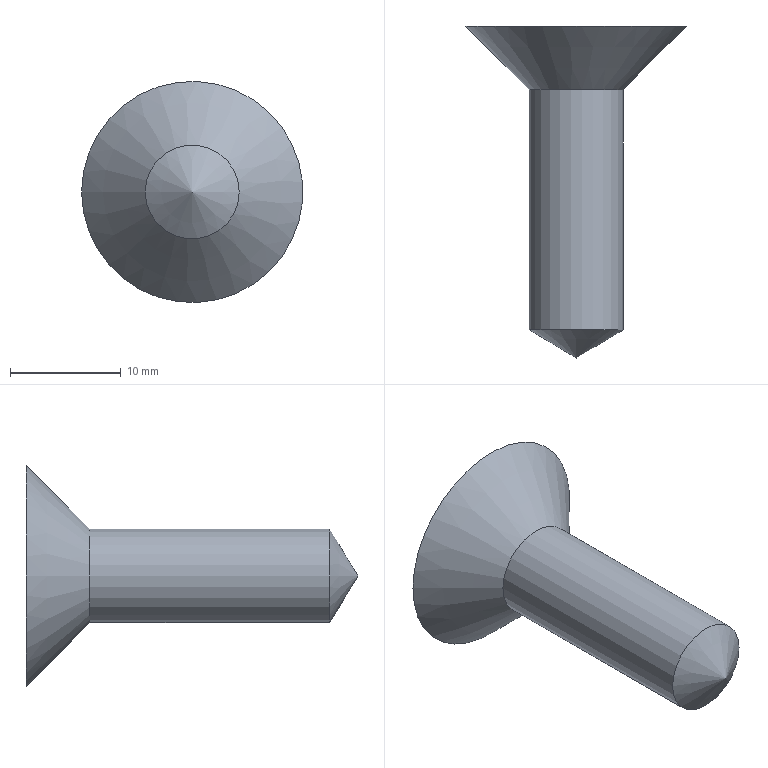Component | NX | SCREW | 1 solid | 17 faces | volume 2186 mm3 | plane 14 | cone 2 | cylinder 1 | commonest cylinder face diameters 8.5 x1